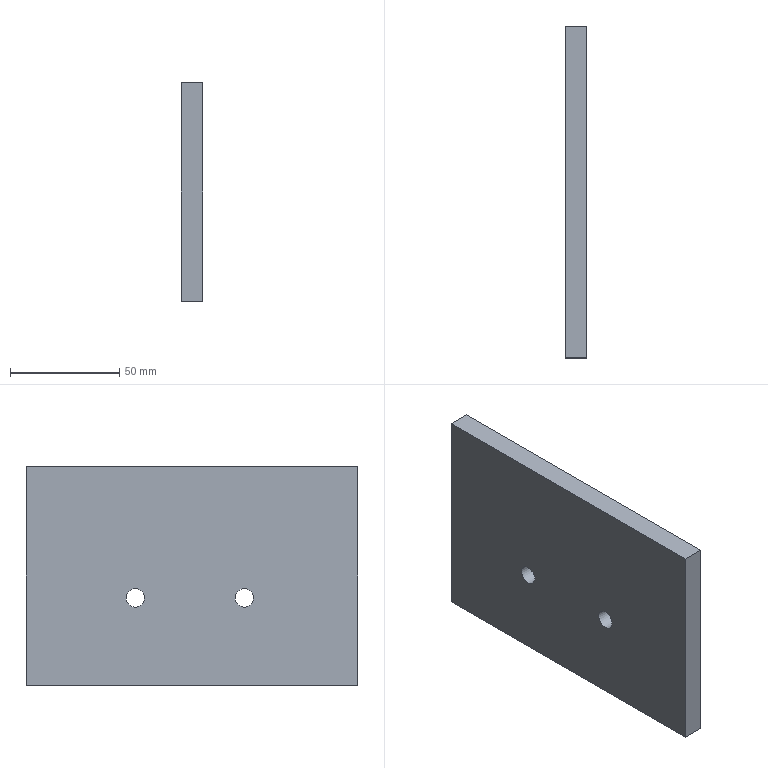Component | NX | FIXED_PLATE_6 | 1 solid | 8 faces | box 10 x 152 x 100 mm | volume 150865 mm3 | plane 6 | cylinder 2 | commonest cylinder face diameters 8.5 x2
STEP:
#1=CARTESIAN_POINT('',(0.,0.,0.));
#2=DIRECTION('',(0.,0.,1.));
#3=DIRECTION('',(1.,0.,0.));
#4=AXIS2_PLACEMENT_3D('',#1,#2,#3);
#5=CARTESIAN_POINT('',(1429.254,1178.,771.574));
#6=VERTEX_POINT('',#5);
#7=CARTESIAN_POINT('',(1429.254,1178.,671.574));
#8=VERTEX_POINT('',#7);
#9=CARTESIAN_POINT('',(1429.254,1178.,771.574));
#10=DIRECTION('',(0.,-0.,-1.));
#11=VECTOR('',#10,1.);
#12=LINE('',#9,#11);
#13=CARTESIAN_POINT('',(1419.254,1178.,771.574));
#14=DIRECTION('',(0.,-1.,0.));
#15=DIRECTION('',(0.,-0.,-1.));
#16=AXIS2_PLACEMENT_3D('',#13,#14,#15);
#17=PLANE('',#16);
#18=CARTESIAN_POINT('',(0.,10.));
#19=DIRECTION('',(1.,0.));
#20=VECTOR('',#19,1.);
#21=LINE('',#18,#20);
#22=(GEOMETRIC_REPRESENTATION_CONTEXT(2)PARAMETRIC_REPRESENTATION_CONTEXT()REPRESENTATION_CONTEXT('',''));
#23=DEFINITIONAL_REPRESENTATION('',(#21),#22);
#24=PCURVE('',#17,#23);
#25=CARTESIAN_POINT('',(1429.254,1230.,711.574));
#26=DIRECTION('',(1.,0.,0.));
#27=DIRECTION('',(0.,0.,-1.));
#28=AXIS2_PLACEMENT_3D('',#25,#26,#27);
#29=PLANE('',#28);
#30=CARTESIAN_POINT('',(-60.,-52.));
#31=DIRECTION('',(1.,-0.));
#32=VECTOR('',#31,1.);
#33=LINE('',#30,#32);
#34=(GEOMETRIC_REPRESENTATION_CONTEXT(2)PARAMETRIC_REPRESENTATION_CONTEXT()REPRESENTATION_CONTEXT('',''));
#35=DEFINITIONAL_REPRESENTATION('',(#33),#34);
#36=PCURVE('',#29,#35);
#37=SURFACE_CURVE('',#12,(#24,#36),.PCURVE_S1.);
#38=EDGE_CURVE('',#6,#8,#37,.T.);
#39=ORIENTED_EDGE('',*,*,#38,.F.);
#40=CARTESIAN_POINT('',(1419.254,1178.,771.574));
#41=VERTEX_POINT('',#40);
#42=CARTESIAN_POINT('',(1419.254,1178.,771.574));
#43=DIRECTION('',(1.,0.,0.));
#44=VECTOR('',#43,1.);
#45=LINE('',#42,#44);
#46=CARTESIAN_POINT('',(0.,0.));
#47=DIRECTION('',(0.,1.));
#48=VECTOR('',#47,1.);
#49=LINE('',#46,#48);
#50=(GEOMETRIC_REPRESENTATION_CONTEXT(2)PARAMETRIC_REPRESENTATION_CONTEXT()REPRESENTATION_CONTEXT('',''));
#51=DEFINITIONAL_REPRESENTATION('',(#49),#50);
#52=PCURVE('',#17,#51);
#53=CARTESIAN_POINT('',(1419.254,1330.,771.574));
#54=DIRECTION('',(0.,0.,1.));
#55=DIRECTION('',(0.,-1.,0.));
#56=AXIS2_PLACEMENT_3D('',#53,#54,#55);
#57=PLANE('',#56);
#58=CARTESIAN_POINT('',(152.,0.));
#59=DIRECTION('',(0.,1.));
#60=VECTOR('',#59,1.);
#61=LINE('',#58,#60);
#62=(GEOMETRIC_REPRESENTATION_CONTEXT(2)PARAMETRIC_REPRESENTATION_CONTEXT()REPRESENTATION_CONTEXT('',''));
#63=DEFINITIONAL_REPRESENTATION('',(#61),#62);
#64=PCURVE('',#57,#63);
#65=SURFACE_CURVE('',#45,(#52,#64),.PCURVE_S1.);
#66=EDGE_CURVE('',#41,#6,#65,.T.);
#67=ORIENTED_EDGE('',*,*,#66,.F.);
#68=CARTESIAN_POINT('',(1419.254,1178.,671.574));
#69=VERTEX_POINT('',#68);
#70=CARTESIAN_POINT('',(1419.254,1178.,771.574));
#71=DIRECTION('',(0.,-0.,-1.));
#72=VECTOR('',#71,1.);
#73=LINE('',#70,#72);
#74=CARTESIAN_POINT('',(0.,0.));
#75=DIRECTION('',(1.,0.));
#76=VECTOR('',#75,1.);
#77=LINE('',#74,#76);
#78=(GEOMETRIC_REPRESENTATION_CONTEXT(2)PARAMETRIC_REPRESENTATION_CONTEXT()REPRESENTATION_CONTEXT('',''));
#79=DEFINITIONAL_REPRESENTATION('',(#77),#78);
#80=PCURVE('',#17,#79);
#81=CARTESIAN_POINT('',(1419.254,1230.,711.574));
#82=DIRECTION('',(1.,0.,0.));
#83=DIRECTION('',(0.,0.,-1.));
#84=AXIS2_PLACEMENT_3D('',#81,#82,#83);
#85=PLANE('',#84);
#86=CARTESIAN_POINT('',(-60.,-52.));
#87=DIRECTION('',(1.,-0.));
#88=VECTOR('',#87,1.);
#89=LINE('',#86,#88);
#90=(GEOMETRIC_REPRESENTATION_CONTEXT(2)PARAMETRIC_REPRESENTATION_CONTEXT()REPRESENTATION_CONTEXT('',''));
#91=DEFINITIONAL_REPRESENTATION('',(#89),#90);
#92=PCURVE('',#85,#91);
#93=SURFACE_CURVE('',#73,(#80,#92),.PCURVE_S1.);
#94=EDGE_CURVE('',#41,#69,#93,.T.);
#95=ORIENTED_EDGE('',*,*,#94,.T.);
#96=CARTESIAN_POINT('',(1419.254,1178.,671.574));
#97=DIRECTION('',(1.,0.,0.));
#98=VECTOR('',#97,1.);
#99=LINE('',#96,#98);
#100=CARTESIAN_POINT('',(100.,0.));
#101=DIRECTION('',(0.,1.));
#102=VECTOR('',#101,1.);
#103=LINE('',#100,#102);
#104=(GEOMETRIC_REPRESENTATION_CONTEXT(2)PARAMETRIC_REPRESENTATION_CONTEXT()REPRESENTATION_CONTEXT('',''));
#105=DEFINITIONAL_REPRESENTATION('',(#103),#104);
#106=PCURVE('',#17,#105);
#107=CARTESIAN_POINT('',(1419.254,1178.,671.574));
#108=DIRECTION('',(0.,0.,-1.));
#109=DIRECTION('',(-1.,0.,0.));
#110=AXIS2_PLACEMENT_3D('',#107,#108,#109);
#111=PLANE('',#110);
#112=CARTESIAN_POINT('',(0.,0.));
#113=DIRECTION('',(-1.,0.));
#114=VECTOR('',#113,1.);
#115=LINE('',#112,#114);
#116=(GEOMETRIC_REPRESENTATION_CONTEXT(2)PARAMETRIC_REPRESENTATION_CONTEXT()REPRESENTATION_CONTEXT('',''));
#117=DEFINITIONAL_REPRESENTATION('',(#115),#116);
#118=PCURVE('',#111,#117);
#119=SURFACE_CURVE('',#99,(#106,#118),.PCURVE_S1.);
#120=EDGE_CURVE('',#69,#8,#119,.T.);
#121=ORIENTED_EDGE('',*,*,#120,.T.);
#122=EDGE_LOOP('',(#39,#67,#95,#121));
#123=FACE_BOUND('',#122,.T.);
#124=ADVANCED_FACE('',(#123),#17,.T.);
#125=CARTESIAN_POINT('',(1429.254,1330.,671.574));
#126=VERTEX_POINT('',#125);
#127=CARTESIAN_POINT('',(1429.254,1178.,671.574));
#128=DIRECTION('',(0.,1.,0.));
#129=VECTOR('',#128,1.);
#130=LINE('',#127,#129);
#131=CARTESIAN_POINT('',(-10.,0.));
#132=DIRECTION('',(0.,1.));
#133=VECTOR('',#132,1.);
#134=LINE('',#131,#133);
#135=(GEOMETRIC_REPRESENTATION_CONTEXT(2)PARAMETRIC_REPRESENTATION_CONTEXT()REPRESENTATION_CONTEXT('',''));
#136=DEFINITIONAL_REPRESENTATION('',(#134),#135);
#137=PCURVE('',#111,#136);
#138=CARTESIAN_POINT('',(40.,-52.));
#139=DIRECTION('',(0.,1.));
#140=VECTOR('',#139,1.);
#141=LINE('',#138,#140);
#142=(GEOMETRIC_REPRESENTATION_CONTEXT(2)PARAMETRIC_REPRESENTATION_CONTEXT()REPRESENTATION_CONTEXT('',''));
#143=DEFINITIONAL_REPRESENTATION('',(#141),#142);
#144=PCURVE('',#29,#143);
#145=SURFACE_CURVE('',#130,(#137,#144),.PCURVE_S1.);
#146=EDGE_CURVE('',#8,#126,#145,.T.);
#147=ORIENTED_EDGE('',*,*,#146,.F.);
#148=ORIENTED_EDGE('',*,*,#120,.F.);
#149=CARTESIAN_POINT('',(1419.254,1330.,671.574));
#150=VERTEX_POINT('',#149);
#151=CARTESIAN_POINT('',(1419.254,1178.,671.574));
#152=DIRECTION('',(0.,1.,0.));
#153=VECTOR('',#152,1.);
#154=LINE('',#151,#153);
#155=CARTESIAN_POINT('',(0.,0.));
#156=DIRECTION('',(0.,1.));
#157=VECTOR('',#156,1.);
#158=LINE('',#155,#157);
#159=(GEOMETRIC_REPRESENTATION_CONTEXT(2)PARAMETRIC_REPRESENTATION_CONTEXT()REPRESENTATION_CONTEXT('',''));
#160=DEFINITIONAL_REPRESENTATION('',(#158),#159);
#161=PCURVE('',#111,#160);
#162=CARTESIAN_POINT('',(40.,-52.));
#163=DIRECTION('',(0.,1.));
#164=VECTOR('',#163,1.);
#165=LINE('',#162,#164);
#166=(GEOMETRIC_REPRESENTATION_CONTEXT(2)PARAMETRIC_REPRESENTATION_CONTEXT()REPRESENTATION_CONTEXT('',''));
#167=DEFINITIONAL_REPRESENTATION('',(#165),#166);
#168=PCURVE('',#85,#167);
#169=SURFACE_CURVE('',#154,(#161,#168),.PCURVE_S1.);
#170=EDGE_CURVE('',#69,#150,#169,.T.);
#171=ORIENTED_EDGE('',*,*,#170,.T.);
#172=CARTESIAN_POINT('',(1419.254,1330.,671.574));
#173=DIRECTION('',(1.,0.,0.));
#174=VECTOR('',#173,1.);
#175=LINE('',#172,#174);
#176=CARTESIAN_POINT('',(0.,152.));
#177=DIRECTION('',(-1.,0.));
#178=VECTOR('',#177,1.);
#179=LINE('',#176,#178);
#180=(GEOMETRIC_REPRESENTATION_CONTEXT(2)PARAMETRIC_REPRESENTATION_CONTEXT()REPRESENTATION_CONTEXT('',''));
#181=DEFINITIONAL_REPRESENTATION('',(#179),#180);
#182=PCURVE('',#111,#181);
#183=CARTESIAN_POINT('',(1419.254,1330.,671.574));
#184=DIRECTION('',(0.,1.,0.));
#185=DIRECTION('',(0.,0.,1.));
#186=AXIS2_PLACEMENT_3D('',#183,#184,#185);
#187=PLANE('',#186);
#188=CARTESIAN_POINT('',(0.,0.));
#189=DIRECTION('',(0.,1.));
#190=VECTOR('',#189,1.);
#191=LINE('',#188,#190);
#192=(GEOMETRIC_REPRESENTATION_CONTEXT(2)PARAMETRIC_REPRESENTATION_CONTEXT()REPRESENTATION_CONTEXT('',''));
#193=DEFINITIONAL_REPRESENTATION('',(#191),#192);
#194=PCURVE('',#187,#193);
#195=SURFACE_CURVE('',#175,(#182,#194),.PCURVE_S1.);
#196=EDGE_CURVE('',#150,#126,#195,.T.);
#197=ORIENTED_EDGE('',*,*,#196,.T.);
#198=EDGE_LOOP('',(#147,#148,#171,#197));
#199=FACE_BOUND('',#198,.T.);
#200=ADVANCED_FACE('',(#199),#111,.T.);
#201=CARTESIAN_POINT('',(1429.254,1330.,771.574));
#202=VERTEX_POINT('',#201);
#203=CARTESIAN_POINT('',(1429.254,1330.,671.574));
#204=DIRECTION('',(0.,0.,1.));
#205=VECTOR('',#204,1.);
#206=LINE('',#203,#205);
#207=CARTESIAN_POINT('',(0.,10.));
#208=DIRECTION('',(1.,0.));
#209=VECTOR('',#208,1.);
#210=LINE('',#207,#209);
#211=(GEOMETRIC_REPRESENTATION_CONTEXT(2)PARAMETRIC_REPRESENTATION_CONTEXT()REPRESENTATION_CONTEXT('',''));
#212=DEFINITIONAL_REPRESENTATION('',(#210),#211);
#213=PCURVE('',#187,#212);
#214=CARTESIAN_POINT('',(40.,100.));
#215=DIRECTION('',(-1.,0.));
#216=VECTOR('',#215,1.);
#217=LINE('',#214,#216);
#218=(GEOMETRIC_REPRESENTATION_CONTEXT(2)PARAMETRIC_REPRESENTATION_CONTEXT()REPRESENTATION_CONTEXT('',''));
#219=DEFINITIONAL_REPRESENTATION('',(#217),#218);
#220=PCURVE('',#29,#219);
#221=SURFACE_CURVE('',#206,(#213,#220),.PCURVE_S1.);
#222=EDGE_CURVE('',#126,#202,#221,.T.);
#223=ORIENTED_EDGE('',*,*,#222,.F.);
#224=ORIENTED_EDGE('',*,*,#196,.F.);
#225=CARTESIAN_POINT('',(1419.254,1330.,771.574));
#226=VERTEX_POINT('',#225);
#227=CARTESIAN_POINT('',(1419.254,1330.,671.574));
#228=DIRECTION('',(0.,0.,1.));
#229=VECTOR('',#228,1.);
#230=LINE('',#227,#229);
#231=CARTESIAN_POINT('',(0.,0.));
#232=DIRECTION('',(1.,0.));
#233=VECTOR('',#232,1.);
#234=LINE('',#231,#233);
#235=(GEOMETRIC_REPRESENTATION_CONTEXT(2)PARAMETRIC_REPRESENTATION_CONTEXT()REPRESENTATION_CONTEXT('',''));
#236=DEFINITIONAL_REPRESENTATION('',(#234),#235);
#237=PCURVE('',#187,#236);
#238=CARTESIAN_POINT('',(40.,100.));
#239=DIRECTION('',(-1.,0.));
#240=VECTOR('',#239,1.);
#241=LINE('',#238,#240);
#242=(GEOMETRIC_REPRESENTATION_CONTEXT(2)PARAMETRIC_REPRESENTATION_CONTEXT()REPRESENTATION_CONTEXT('',''));
#243=DEFINITIONAL_REPRESENTATION('',(#241),#242);
#244=PCURVE('',#85,#243);
#245=SURFACE_CURVE('',#230,(#237,#244),.PCURVE_S1.);
#246=EDGE_CURVE('',#150,#226,#245,.T.);
#247=ORIENTED_EDGE('',*,*,#246,.T.);
#248=CARTESIAN_POINT('',(1419.254,1330.,771.574));
#249=DIRECTION('',(1.,0.,0.));
#250=VECTOR('',#249,1.);
#251=LINE('',#248,#250);
#252=CARTESIAN_POINT('',(100.,0.));
#253=DIRECTION('',(0.,1.));
#254=VECTOR('',#253,1.);
#255=LINE('',#252,#254);
#256=(GEOMETRIC_REPRESENTATION_CONTEXT(2)PARAMETRIC_REPRESENTATION_CONTEXT()REPRESENTATION_CONTEXT('',''));
#257=DEFINITIONAL_REPRESENTATION('',(#255),#256);
#258=PCURVE('',#187,#257);
#259=CARTESIAN_POINT('',(0.,0.));
#260=DIRECTION('',(0.,1.));
#261=VECTOR('',#260,1.);
#262=LINE('',#259,#261);
#263=(GEOMETRIC_REPRESENTATION_CONTEXT(2)PARAMETRIC_REPRESENTATION_CONTEXT()REPRESENTATION_CONTEXT('',''));
#264=DEFINITIONAL_REPRESENTATION('',(#262),#263);
#265=PCURVE('',#57,#264);
#266=SURFACE_CURVE('',#251,(#258,#265),.PCURVE_S1.);
#267=EDGE_CURVE('',#226,#202,#266,.T.);
#268=ORIENTED_EDGE('',*,*,#267,.T.);
#269=EDGE_LOOP('',(#223,#224,#247,#268));
#270=FACE_BOUND('',#269,.T.);
#271=ADVANCED_FACE('',(#270),#187,.T.);
#272=CARTESIAN_POINT('',(1419.254,1234.25,711.574));
#273=VERTEX_POINT('',#272);
#274=CARTESIAN_POINT('',(1419.254,1230.,711.574));
#275=DIRECTION('',(1.,0.,0.));
#276=DIRECTION('',(0.,1.,0.));
#277=AXIS2_PLACEMENT_3D('',#274,#275,#276);
#278=CIRCLE('',#277,4.25);
#279=CARTESIAN_POINT('',(1419.254,1230.,711.574));
#280=DIRECTION('',(1.,0.,0.));
#281=DIRECTION('',(0.,0.,-1.));
#282=AXIS2_PLACEMENT_3D('',#279,#280,#281);
#283=CYLINDRICAL_SURFACE('',#282,4.25);
#284=CARTESIAN_POINT('',(1.571,0.));
#285=DIRECTION('',(1.,0.));
#286=VECTOR('',#285,1.);
#287=LINE('',#284,#286);
#288=(GEOMETRIC_REPRESENTATION_CONTEXT(2)PARAMETRIC_REPRESENTATION_CONTEXT()REPRESENTATION_CONTEXT('',''));
#289=DEFINITIONAL_REPRESENTATION('',(#287),#288);
#290=PCURVE('',#283,#289);
#291=CARTESIAN_POINT('',(0.,0.));
#292=DIRECTION('',(0.,1.));
#293=AXIS2_PLACEMENT_2D('',#291,#292);
#294=CIRCLE('',#293,4.25);
#295=(GEOMETRIC_REPRESENTATION_CONTEXT(2)PARAMETRIC_REPRESENTATION_CONTEXT()REPRESENTATION_CONTEXT('',''));
#296=DEFINITIONAL_REPRESENTATION('',(#294),#295);
#297=PCURVE('',#85,#296);
#298=SURFACE_CURVE('',#278,(#290,#297),.PCURVE_S1.);
#299=EDGE_CURVE('',#273,#273,#298,.T.);
#300=ORIENTED_EDGE('',*,*,#299,.T.);
#301=CARTESIAN_POINT('',(1429.254,1234.25,711.574));
#302=VERTEX_POINT('',#301);
#303=CARTESIAN_POINT('',(1419.254,1234.25,711.574));
#304=CARTESIAN_POINT('',(1429.254,1234.25,711.574));
#305=B_SPLINE_CURVE_WITH_KNOTS('',1,(#303,#304),.UNSPECIFIED.,.F.,.F.,(2,2),(0.,10.),.PIECEWISE_BEZIER_KNOTS.);
#306=CARTESIAN_POINT('',(7.854,0.));
#307=DIRECTION('',(0.,1.));
#308=VECTOR('',#307,1.);
#309=LINE('',#306,#308);
#310=(GEOMETRIC_REPRESENTATION_CONTEXT(2)PARAMETRIC_REPRESENTATION_CONTEXT()REPRESENTATION_CONTEXT('',''));
#311=DEFINITIONAL_REPRESENTATION('',(#309),#310);
#312=PCURVE('',#283,#311);
#313=CARTESIAN_POINT('',(1.571,0.));
#314=DIRECTION('',(0.,1.));
#315=VECTOR('',#314,1.);
#316=LINE('',#313,#315);
#317=(GEOMETRIC_REPRESENTATION_CONTEXT(2)PARAMETRIC_REPRESENTATION_CONTEXT()REPRESENTATION_CONTEXT('',''));
#318=DEFINITIONAL_REPRESENTATION('',(#316),#317);
#319=PCURVE('',#283,#318);
#320=SEAM_CURVE('',#305,(#312,#319),.PCURVE_S1.);
#321=EDGE_CURVE('',#273,#302,#320,.T.);
#322=ORIENTED_EDGE('',*,*,#321,.T.);
#323=CARTESIAN_POINT('',(1429.254,1230.,711.574));
#324=DIRECTION('',(1.,0.,0.));
#325=DIRECTION('',(0.,1.,0.));
#326=AXIS2_PLACEMENT_3D('',#323,#324,#325);
#327=CIRCLE('',#326,4.25);
#328=CARTESIAN_POINT('',(1.571,10.));
#329=DIRECTION('',(1.,0.));
#330=VECTOR('',#329,1.);
#331=LINE('',#328,#330);
#332=(GEOMETRIC_REPRESENTATION_CONTEXT(2)PARAMETRIC_REPRESENTATION_CONTEXT()REPRESENTATION_CONTEXT('',''));
#333=DEFINITIONAL_REPRESENTATION('',(#331),#332);
#334=PCURVE('',#283,#333);
#335=CARTESIAN_POINT('',(0.,0.));
#336=DIRECTION('',(0.,1.));
#337=AXIS2_PLACEMENT_2D('',#335,#336);
#338=CIRCLE('',#337,4.25);
#339=(GEOMETRIC_REPRESENTATION_CONTEXT(2)PARAMETRIC_REPRESENTATION_CONTEXT()REPRESENTATION_CONTEXT('',''));
#340=DEFINITIONAL_REPRESENTATION('',(#338),#339);
#341=PCURVE('',#29,#340);
#342=SURFACE_CURVE('',#327,(#334,#341),.PCURVE_S1.);
#343=EDGE_CURVE('',#302,#302,#342,.T.);
#344=ORIENTED_EDGE('',*,*,#343,.F.);
#345=ORIENTED_EDGE('',*,*,#321,.F.);
#346=EDGE_LOOP('',(#300,#322,#344,#345));
#347=FACE_BOUND('',#346,.F.);
#348=ADVANCED_FACE('',(#347),#283,.F.);
#349=CARTESIAN_POINT('',(1429.254,1330.,771.574));
#350=DIRECTION('',(0.,-1.,0.));
#351=VECTOR('',#350,1.);
#352=LINE('',#349,#351);
#353=CARTESIAN_POINT('',(0.,10.));
#354=DIRECTION('',(1.,0.));
#355=VECTOR('',#354,1.);
#356=LINE('',#353,#355);
#357=(GEOMETRIC_REPRESENTATION_CONTEXT(2)PARAMETRIC_REPRESENTATION_CONTEXT()REPRESENTATION_CONTEXT('',''));
#358=DEFINITIONAL_REPRESENTATION('',(#356),#357);
#359=PCURVE('',#57,#358);
#360=CARTESIAN_POINT('',(-60.,100.));
#361=DIRECTION('',(-0.,-1.));
#362=VECTOR('',#361,1.);
#363=LINE('',#360,#362);
#364=(GEOMETRIC_REPRESENTATION_CONTEXT(2)PARAMETRIC_REPRESENTATION_CONTEXT()REPRESENTATION_CONTEXT('',''));
#365=DEFINITIONAL_REPRESENTATION('',(#363),#364);
#366=PCURVE('',#29,#365);
#367=SURFACE_CURVE('',#352,(#359,#366),.PCURVE_S1.);
#368=EDGE_CURVE('',#202,#6,#367,.T.);
#369=ORIENTED_EDGE('',*,*,#368,.F.);
#370=ORIENTED_EDGE('',*,*,#267,.F.);
#371=CARTESIAN_POINT('',(1419.254,1330.,771.574));
#372=DIRECTION('',(0.,-1.,0.));
#373=VECTOR('',#372,1.);
#374=LINE('',#371,#373);
#375=CARTESIAN_POINT('',(0.,0.));
#376=DIRECTION('',(1.,0.));
#377=VECTOR('',#376,1.);
#378=LINE('',#375,#377);
#379=(GEOMETRIC_REPRESENTATION_CONTEXT(2)PARAMETRIC_REPRESENTATION_CONTEXT()REPRESENTATION_CONTEXT('',''));
#380=DEFINITIONAL_REPRESENTATION('',(#378),#379);
#381=PCURVE('',#57,#380);
#382=CARTESIAN_POINT('',(-60.,100.));
#383=DIRECTION('',(-0.,-1.));
#384=VECTOR('',#383,1.);
#385=LINE('',#382,#384);
#386=(GEOMETRIC_REPRESENTATION_CONTEXT(2)PARAMETRIC_REPRESENTATION_CONTEXT()REPRESENTATION_CONTEXT('',''));
#387=DEFINITIONAL_REPRESENTATION('',(#385),#386);
#388=PCURVE('',#85,#387);
#389=SURFACE_CURVE('',#374,(#381,#388),.PCURVE_S1.);
#390=EDGE_CURVE('',#226,#41,#389,.T.);
#391=ORIENTED_EDGE('',*,*,#390,.T.);
#392=ORIENTED_EDGE('',*,*,#66,.T.);
#393=EDGE_LOOP('',(#369,#370,#391,#392));
#394=FACE_BOUND('',#393,.T.);
#395=ADVANCED_FACE('',(#394),#57,.T.);
#396=CARTESIAN_POINT('',(1419.254,1284.25,711.574));
#397=VERTEX_POINT('',#396);
#398=CARTESIAN_POINT('',(1419.254,1280.,711.574));
#399=DIRECTION('',(1.,0.,0.));
#400=DIRECTION('',(0.,1.,0.));
#401=AXIS2_PLACEMENT_3D('',#398,#399,#400);
#402=CIRCLE('',#401,4.25);
#403=CARTESIAN_POINT('',(1419.254,1280.,711.574));
#404=DIRECTION('',(1.,0.,0.));
#405=DIRECTION('',(0.,0.,-1.));
#406=AXIS2_PLACEMENT_3D('',#403,#404,#405);
#407=CYLINDRICAL_SURFACE('',#406,4.25);
#408=CARTESIAN_POINT('',(1.571,0.));
#409=DIRECTION('',(1.,0.));
#410=VECTOR('',#409,1.);
#411=LINE('',#408,#410);
#412=(GEOMETRIC_REPRESENTATION_CONTEXT(2)PARAMETRIC_REPRESENTATION_CONTEXT()REPRESENTATION_CONTEXT('',''));
#413=DEFINITIONAL_REPRESENTATION('',(#411),#412);
#414=PCURVE('',#407,#413);
#415=CARTESIAN_POINT('',(0.,50.));
#416=DIRECTION('',(0.,1.));
#417=AXIS2_PLACEMENT_2D('',#415,#416);
#418=CIRCLE('',#417,4.25);
#419=(GEOMETRIC_REPRESENTATION_CONTEXT(2)PARAMETRIC_REPRESENTATION_CONTEXT()REPRESENTATION_CONTEXT('',''));
#420=DEFINITIONAL_REPRESENTATION('',(#418),#419);
#421=PCURVE('',#85,#420);
#422=SURFACE_CURVE('',#402,(#414,#421),.PCURVE_S1.);
#423=EDGE_CURVE('',#397,#397,#422,.T.);
#424=ORIENTED_EDGE('',*,*,#423,.T.);
#425=CARTESIAN_POINT('',(1429.254,1284.25,711.574));
#426=VERTEX_POINT('',#425);
#427=CARTESIAN_POINT('',(1419.254,1284.25,711.574));
#428=CARTESIAN_POINT('',(1429.254,1284.25,711.574));
#429=B_SPLINE_CURVE_WITH_KNOTS('',1,(#427,#428),.UNSPECIFIED.,.F.,.F.,(2,2),(0.,10.),.PIECEWISE_BEZIER_KNOTS.);
#430=CARTESIAN_POINT('',(7.854,0.));
#431=DIRECTION('',(0.,1.));
#432=VECTOR('',#431,1.);
#433=LINE('',#430,#432);
#434=(GEOMETRIC_REPRESENTATION_CONTEXT(2)PARAMETRIC_REPRESENTATION_CONTEXT()REPRESENTATION_CONTEXT('',''));
#435=DEFINITIONAL_REPRESENTATION('',(#433),#434);
#436=PCURVE('',#407,#435);
#437=CARTESIAN_POINT('',(1.571,0.));
#438=DIRECTION('',(0.,1.));
#439=VECTOR('',#438,1.);
#440=LINE('',#437,#439);
#441=(GEOMETRIC_REPRESENTATION_CONTEXT(2)PARAMETRIC_REPRESENTATION_CONTEXT()REPRESENTATION_CONTEXT('',''));
#442=DEFINITIONAL_REPRESENTATION('',(#440),#441);
#443=PCURVE('',#407,#442);
#444=SEAM_CURVE('',#429,(#436,#443),.PCURVE_S1.);
#445=EDGE_CURVE('',#397,#426,#444,.T.);
#446=ORIENTED_EDGE('',*,*,#445,.T.);
#447=CARTESIAN_POINT('',(1429.254,1280.,711.574));
#448=DIRECTION('',(1.,0.,0.));
#449=DIRECTION('',(0.,1.,0.));
#450=AXIS2_PLACEMENT_3D('',#447,#448,#449);
#451=CIRCLE('',#450,4.25);
#452=CARTESIAN_POINT('',(1.571,10.));
#453=DIRECTION('',(1.,0.));
#454=VECTOR('',#453,1.);
#455=LINE('',#452,#454);
#456=(GEOMETRIC_REPRESENTATION_CONTEXT(2)PARAMETRIC_REPRESENTATION_CONTEXT()REPRESENTATION_CONTEXT('',''));
#457=DEFINITIONAL_REPRESENTATION('',(#455),#456);
#458=PCURVE('',#407,#457);
#459=CARTESIAN_POINT('',(0.,50.));
#460=DIRECTION('',(0.,1.));
#461=AXIS2_PLACEMENT_2D('',#459,#460);
#462=CIRCLE('',#461,4.25);
#463=(GEOMETRIC_REPRESENTATION_CONTEXT(2)PARAMETRIC_REPRESENTATION_CONTEXT()REPRESENTATION_CONTEXT('',''));
#464=DEFINITIONAL_REPRESENTATION('',(#462),#463);
#465=PCURVE('',#29,#464);
#466=SURFACE_CURVE('',#451,(#458,#465),.PCURVE_S1.);
#467=EDGE_CURVE('',#426,#426,#466,.T.);
#468=ORIENTED_EDGE('',*,*,#467,.F.);
#469=ORIENTED_EDGE('',*,*,#445,.F.);
#470=EDGE_LOOP('',(#424,#446,#468,#469));
#471=FACE_BOUND('',#470,.F.);
#472=ADVANCED_FACE('',(#471),#407,.F.);
#473=ORIENTED_EDGE('',*,*,#94,.F.);
#474=ORIENTED_EDGE('',*,*,#390,.F.);
#475=ORIENTED_EDGE('',*,*,#246,.F.);
#476=ORIENTED_EDGE('',*,*,#170,.F.);
#477=EDGE_LOOP('',(#473,#474,#475,#476));
#478=FACE_BOUND('',#477,.T.);
#479=ORIENTED_EDGE('',*,*,#299,.T.);
#480=EDGE_LOOP('',(#479));
#481=FACE_BOUND('',#480,.T.);
#482=ORIENTED_EDGE('',*,*,#423,.T.);
#483=EDGE_LOOP('',(#482));
#484=FACE_BOUND('',#483,.T.);
#485=ADVANCED_FACE('',(#478,#481,#484),#85,.F.);
#486=ORIENTED_EDGE('',*,*,#38,.T.);
#487=ORIENTED_EDGE('',*,*,#146,.T.);
#488=ORIENTED_EDGE('',*,*,#222,.T.);
#489=ORIENTED_EDGE('',*,*,#368,.T.);
#490=EDGE_LOOP('',(#486,#487,#488,#489));
#491=FACE_BOUND('',#490,.T.);
#492=ORIENTED_EDGE('',*,*,#343,.F.);
#493=EDGE_LOOP('',(#492));
#494=FACE_BOUND('',#493,.T.);
#495=ORIENTED_EDGE('',*,*,#467,.F.);
#496=EDGE_LOOP('',(#495));
#497=FACE_BOUND('',#496,.T.);
#498=ADVANCED_FACE('',(#491,#494,#497),#29,.T.);
#499=CLOSED_SHELL('',(#124,#200,#271,#348,#395,#472,#485,#498));
#500=MANIFOLD_SOLID_BREP('',#499);
#501=(LENGTH_UNIT()NAMED_UNIT(*)SI_UNIT(.MILLI.,.METRE.));
#502=UNCERTAINTY_MEASURE_WITH_UNIT(LENGTH_MEASURE(0.000002),#501,'','');
#503=(NAMED_UNIT(*)PLANE_ANGLE_UNIT()SI_UNIT($,.RADIAN.));
#504=(NAMED_UNIT(*)SI_UNIT($,.STERADIAN.)SOLID_ANGLE_UNIT());
#505=(GEOMETRIC_REPRESENTATION_CONTEXT(3)GLOBAL_UNCERTAINTY_ASSIGNED_CONTEXT((#502))GLOBAL_UNIT_ASSIGNED_CONTEXT((#501,#503,#504))REPRESENTATION_CONTEXT('',''));
#506=ADVANCED_BREP_SHAPE_REPRESENTATION('',(#4,#500),#505);